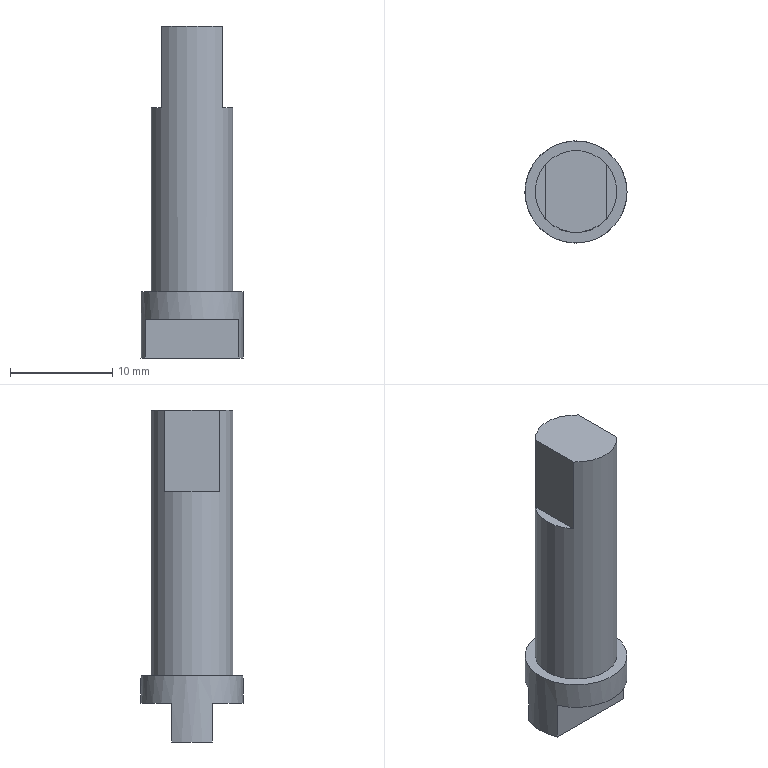Component | NX | VALVE_STEM | 1 solid | 13 faces | box 10 x 10 x 32.5 mm | volume 1609 mm3 | plane 11 | cylinder 2 | commonest cylinder face diameters 10 x1 8 x1
STEP:
#1=CARTESIAN_POINT('',(0.,0.,0.));
#2=DIRECTION('',(0.,0.,1.));
#3=DIRECTION('',(1.,0.,0.));
#4=AXIS2_PLACEMENT_3D('',#1,#2,#3);
#5=CARTESIAN_POINT('',(4.,14.,37.2));
#6=VERTEX_POINT('',#5);
#7=CARTESIAN_POINT('',(0.,14.,37.2));
#8=DIRECTION('',(0.,0.,1.));
#9=DIRECTION('',(1.,0.,0.));
#10=AXIS2_PLACEMENT_3D('',#7,#8,#9);
#11=CIRCLE('',#10,4.);
#12=CARTESIAN_POINT('',(0.,14.,37.2));
#13=DIRECTION('',(0.,0.,1.));
#14=DIRECTION('',(1.,0.,0.));
#15=AXIS2_PLACEMENT_3D('',#12,#13,#14);
#16=PLANE('',#15);
#17=CARTESIAN_POINT('',(0.,0.));
#18=DIRECTION('',(1.,0.));
#19=AXIS2_PLACEMENT_2D('',#17,#18);
#20=CIRCLE('',#19,4.);
#21=(GEOMETRIC_REPRESENTATION_CONTEXT(2)PARAMETRIC_REPRESENTATION_CONTEXT()REPRESENTATION_CONTEXT('',''));
#22=DEFINITIONAL_REPRESENTATION('',(#20),#21);
#23=PCURVE('',#16,#22);
#24=CARTESIAN_POINT('',(0.,14.,37.2));
#25=DIRECTION('',(0.,0.,1.));
#26=DIRECTION('',(1.,0.,0.));
#27=AXIS2_PLACEMENT_3D('',#24,#25,#26);
#28=CYLINDRICAL_SURFACE('',#27,4.);
#29=CARTESIAN_POINT('',(0.,0.));
#30=DIRECTION('',(1.,0.));
#31=VECTOR('',#30,1.);
#32=LINE('',#29,#31);
#33=(GEOMETRIC_REPRESENTATION_CONTEXT(2)PARAMETRIC_REPRESENTATION_CONTEXT()REPRESENTATION_CONTEXT('',''));
#34=DEFINITIONAL_REPRESENTATION('',(#32),#33);
#35=PCURVE('',#28,#34);
#36=SURFACE_CURVE('',#11,(#23,#35),.PCURVE_S1.);
#37=EDGE_CURVE('',#6,#6,#36,.T.);
#38=ORIENTED_EDGE('',*,*,#37,.F.);
#39=EDGE_LOOP('',(#38));
#40=FACE_BOUND('',#39,.T.);
#41=CARTESIAN_POINT('',(5.,14.,37.2));
#42=VERTEX_POINT('',#41);
#43=CARTESIAN_POINT('',(0.,14.,37.2));
#44=DIRECTION('',(0.,0.,-1.));
#45=DIRECTION('',(1.,0.,0.));
#46=AXIS2_PLACEMENT_3D('',#43,#44,#45);
#47=CIRCLE('',#46,5.);
#48=CARTESIAN_POINT('',(5.,0.));
#49=CARTESIAN_POINT('',(5.,-8.66));
#50=CARTESIAN_POINT('',(-2.5,-4.33));
#51=CARTESIAN_POINT('',(-10.,-0.));
#52=CARTESIAN_POINT('',(-2.5,4.33));
#53=CARTESIAN_POINT('',(5.,8.66));
#54=CARTESIAN_POINT('',(5.,0.));
#55=(BOUNDED_CURVE()B_SPLINE_CURVE(2,(#48,#49,#50,#51,#52,#53,#54),.UNSPECIFIED.,.T.,.F.)B_SPLINE_CURVE_WITH_KNOTS((1,2,2,2,2,1),(-2.094,0.,2.094,4.189,6.283,8.378),.UNSPECIFIED.)CURVE()GEOMETRIC_REPRESENTATION_ITEM()RATIONAL_B_SPLINE_CURVE((1.,0.5,1.,0.5,1.,0.5,1.))REPRESENTATION_ITEM(''));
#56=(GEOMETRIC_REPRESENTATION_CONTEXT(2)PARAMETRIC_REPRESENTATION_CONTEXT()REPRESENTATION_CONTEXT('',''));
#57=DEFINITIONAL_REPRESENTATION('',(#55),#56);
#58=PCURVE('',#16,#57);
#59=CARTESIAN_POINT('',(0.,14.,30.7));
#60=DIRECTION('',(0.,0.,1.));
#61=DIRECTION('',(1.,0.,0.));
#62=AXIS2_PLACEMENT_3D('',#59,#60,#61);
#63=CYLINDRICAL_SURFACE('',#62,5.);
#64=CARTESIAN_POINT('',(6.283,6.5));
#65=DIRECTION('',(-1.,0.));
#66=VECTOR('',#65,1.);
#67=LINE('',#64,#66);
#68=(GEOMETRIC_REPRESENTATION_CONTEXT(2)PARAMETRIC_REPRESENTATION_CONTEXT()REPRESENTATION_CONTEXT('',''));
#69=DEFINITIONAL_REPRESENTATION('',(#67),#68);
#70=PCURVE('',#63,#69);
#71=SURFACE_CURVE('',#47,(#58,#70),.PCURVE_S1.);
#72=EDGE_CURVE('',#42,#42,#71,.T.);
#73=ORIENTED_EDGE('',*,*,#72,.F.);
#74=EDGE_LOOP('',(#73));
#75=FACE_BOUND('',#74,.T.);
#76=ADVANCED_FACE('',(#40,#75),#16,.T.);
#77=CARTESIAN_POINT('',(-4.583,12.,30.7));
#78=VERTEX_POINT('',#77);
#79=CARTESIAN_POINT('',(4.583,12.,30.7));
#80=VERTEX_POINT('',#79);
#81=CARTESIAN_POINT('',(0.,12.,30.7));
#82=DIRECTION('',(1.,0.,0.));
#83=VECTOR('',#82,1.);
#84=LINE('',#81,#83);
#85=CARTESIAN_POINT('',(0.,14.,30.7));
#86=DIRECTION('',(0.,0.,-1.));
#87=DIRECTION('',(-1.,0.,0.));
#88=AXIS2_PLACEMENT_3D('',#85,#86,#87);
#89=PLANE('',#88);
#90=CARTESIAN_POINT('',(0.,-2.));
#91=DIRECTION('',(-1.,0.));
#92=VECTOR('',#91,1.);
#93=LINE('',#90,#92);
#94=(GEOMETRIC_REPRESENTATION_CONTEXT(2)PARAMETRIC_REPRESENTATION_CONTEXT()REPRESENTATION_CONTEXT('',''));
#95=DEFINITIONAL_REPRESENTATION('',(#93),#94);
#96=PCURVE('',#89,#95);
#97=CARTESIAN_POINT('',(-10.,12.,29.7));
#98=DIRECTION('',(0.,1.,-0.));
#99=DIRECTION('',(0.,0.,1.));
#100=AXIS2_PLACEMENT_3D('',#97,#98,#99);
#101=PLANE('',#100);
#102=CARTESIAN_POINT('',(1.,10.));
#103=DIRECTION('',(0.,1.));
#104=VECTOR('',#103,1.);
#105=LINE('',#102,#104);
#106=(GEOMETRIC_REPRESENTATION_CONTEXT(2)PARAMETRIC_REPRESENTATION_CONTEXT()REPRESENTATION_CONTEXT('',''));
#107=DEFINITIONAL_REPRESENTATION('',(#105),#106);
#108=PCURVE('',#101,#107);
#109=SURFACE_CURVE('',#84,(#96,#108),.PCURVE_S1.);
#110=EDGE_CURVE('',#78,#80,#109,.T.);
#111=ORIENTED_EDGE('',*,*,#110,.F.);
#112=CARTESIAN_POINT('',(-4.583,16.,30.7));
#113=VERTEX_POINT('',#112);
#114=CARTESIAN_POINT('',(0.,14.,30.7));
#115=DIRECTION('',(0.,0.,1.));
#116=DIRECTION('',(1.,0.,0.));
#117=AXIS2_PLACEMENT_3D('',#114,#115,#116);
#118=CIRCLE('',#117,5.);
#119=CARTESIAN_POINT('',(-5.,0.));
#120=CARTESIAN_POINT('',(-5.,8.66));
#121=CARTESIAN_POINT('',(2.5,4.33));
#122=CARTESIAN_POINT('',(10.,0.));
#123=CARTESIAN_POINT('',(2.5,-4.33));
#124=CARTESIAN_POINT('',(-5.,-8.66));
#125=CARTESIAN_POINT('',(-5.,0.));
#126=(BOUNDED_CURVE()B_SPLINE_CURVE(2,(#119,#120,#121,#122,#123,#124,#125),.UNSPECIFIED.,.T.,.F.)B_SPLINE_CURVE_WITH_KNOTS((1,2,2,2,2,1),(-2.094,0.,2.094,4.189,6.283,8.378),.UNSPECIFIED.)CURVE()GEOMETRIC_REPRESENTATION_ITEM()RATIONAL_B_SPLINE_CURVE((1.,0.5,1.,0.5,1.,0.5,1.))REPRESENTATION_ITEM(''));
#127=(GEOMETRIC_REPRESENTATION_CONTEXT(2)PARAMETRIC_REPRESENTATION_CONTEXT()REPRESENTATION_CONTEXT('',''));
#128=DEFINITIONAL_REPRESENTATION('',(#126),#127);
#129=PCURVE('',#89,#128);
#130=CARTESIAN_POINT('',(0.,0.));
#131=DIRECTION('',(1.,0.));
#132=VECTOR('',#131,1.);
#133=LINE('',#130,#132);
#134=(GEOMETRIC_REPRESENTATION_CONTEXT(2)PARAMETRIC_REPRESENTATION_CONTEXT()REPRESENTATION_CONTEXT('',''));
#135=DEFINITIONAL_REPRESENTATION('',(#133),#134);
#136=PCURVE('',#63,#135);
#137=SURFACE_CURVE('',#118,(#129,#136),.PCURVE_S1.);
#138=EDGE_CURVE('',#113,#78,#137,.T.);
#139=ORIENTED_EDGE('',*,*,#138,.F.);
#140=CARTESIAN_POINT('',(4.583,16.,30.7));
#141=VERTEX_POINT('',#140);
#142=CARTESIAN_POINT('',(0.,16.,30.7));
#143=DIRECTION('',(-1.,0.,0.));
#144=VECTOR('',#143,1.);
#145=LINE('',#142,#144);
#146=CARTESIAN_POINT('',(0.,2.));
#147=DIRECTION('',(1.,0.));
#148=VECTOR('',#147,1.);
#149=LINE('',#146,#148);
#150=(GEOMETRIC_REPRESENTATION_CONTEXT(2)PARAMETRIC_REPRESENTATION_CONTEXT()REPRESENTATION_CONTEXT('',''));
#151=DEFINITIONAL_REPRESENTATION('',(#149),#150);
#152=PCURVE('',#89,#151);
#153=CARTESIAN_POINT('',(-10.,16.,34.5));
#154=DIRECTION('',(0.,-1.,-0.));
#155=DIRECTION('',(0.,0.,-1.));
#156=AXIS2_PLACEMENT_3D('',#153,#154,#155);
#157=PLANE('',#156);
#158=CARTESIAN_POINT('',(3.8,10.));
#159=DIRECTION('',(0.,-1.));
#160=VECTOR('',#159,1.);
#161=LINE('',#158,#160);
#162=(GEOMETRIC_REPRESENTATION_CONTEXT(2)PARAMETRIC_REPRESENTATION_CONTEXT()REPRESENTATION_CONTEXT('',''));
#163=DEFINITIONAL_REPRESENTATION('',(#161),#162);
#164=PCURVE('',#157,#163);
#165=SURFACE_CURVE('',#145,(#152,#164),.PCURVE_S1.);
#166=EDGE_CURVE('',#141,#113,#165,.T.);
#167=ORIENTED_EDGE('',*,*,#166,.F.);
#168=CARTESIAN_POINT('',(5.,14.,30.7));
#169=VERTEX_POINT('',#168);
#170=CARTESIAN_POINT('',(0.,14.,30.7));
#171=DIRECTION('',(0.,0.,1.));
#172=DIRECTION('',(1.,0.,0.));
#173=AXIS2_PLACEMENT_3D('',#170,#171,#172);
#174=CIRCLE('',#173,5.);
#175=CARTESIAN_POINT('',(-5.,0.));
#176=CARTESIAN_POINT('',(-5.,8.66));
#177=CARTESIAN_POINT('',(2.5,4.33));
#178=CARTESIAN_POINT('',(10.,0.));
#179=CARTESIAN_POINT('',(2.5,-4.33));
#180=CARTESIAN_POINT('',(-5.,-8.66));
#181=CARTESIAN_POINT('',(-5.,0.));
#182=(BOUNDED_CURVE()B_SPLINE_CURVE(2,(#175,#176,#177,#178,#179,#180,#181),.UNSPECIFIED.,.T.,.F.)B_SPLINE_CURVE_WITH_KNOTS((1,2,2,2,2,1),(-2.094,0.,2.094,4.189,6.283,8.378),.UNSPECIFIED.)CURVE()GEOMETRIC_REPRESENTATION_ITEM()RATIONAL_B_SPLINE_CURVE((1.,0.5,1.,0.5,1.,0.5,1.))REPRESENTATION_ITEM(''));
#183=(GEOMETRIC_REPRESENTATION_CONTEXT(2)PARAMETRIC_REPRESENTATION_CONTEXT()REPRESENTATION_CONTEXT('',''));
#184=DEFINITIONAL_REPRESENTATION('',(#182),#183);
#185=PCURVE('',#89,#184);
#186=CARTESIAN_POINT('',(-6.283,0.));
#187=DIRECTION('',(1.,0.));
#188=VECTOR('',#187,1.);
#189=LINE('',#186,#188);
#190=(GEOMETRIC_REPRESENTATION_CONTEXT(2)PARAMETRIC_REPRESENTATION_CONTEXT()REPRESENTATION_CONTEXT('',''));
#191=DEFINITIONAL_REPRESENTATION('',(#189),#190);
#192=PCURVE('',#63,#191);
#193=SURFACE_CURVE('',#174,(#185,#192),.PCURVE_S1.);
#194=EDGE_CURVE('',#169,#141,#193,.T.);
#195=ORIENTED_EDGE('',*,*,#194,.F.);
#196=CARTESIAN_POINT('',(0.,14.,30.7));
#197=DIRECTION('',(0.,0.,1.));
#198=DIRECTION('',(1.,0.,0.));
#199=AXIS2_PLACEMENT_3D('',#196,#197,#198);
#200=CIRCLE('',#199,5.);
#201=CARTESIAN_POINT('',(-5.,0.));
#202=CARTESIAN_POINT('',(-5.,8.66));
#203=CARTESIAN_POINT('',(2.5,4.33));
#204=CARTESIAN_POINT('',(10.,0.));
#205=CARTESIAN_POINT('',(2.5,-4.33));
#206=CARTESIAN_POINT('',(-5.,-8.66));
#207=CARTESIAN_POINT('',(-5.,0.));
#208=(BOUNDED_CURVE()B_SPLINE_CURVE(2,(#201,#202,#203,#204,#205,#206,#207),.UNSPECIFIED.,.T.,.F.)B_SPLINE_CURVE_WITH_KNOTS((1,2,2,2,2,1),(-2.094,0.,2.094,4.189,6.283,8.378),.UNSPECIFIED.)CURVE()GEOMETRIC_REPRESENTATION_ITEM()RATIONAL_B_SPLINE_CURVE((1.,0.5,1.,0.5,1.,0.5,1.))REPRESENTATION_ITEM(''));
#209=(GEOMETRIC_REPRESENTATION_CONTEXT(2)PARAMETRIC_REPRESENTATION_CONTEXT()REPRESENTATION_CONTEXT('',''));
#210=DEFINITIONAL_REPRESENTATION('',(#208),#209);
#211=PCURVE('',#89,#210);
#212=CARTESIAN_POINT('',(0.,0.));
#213=DIRECTION('',(1.,0.));
#214=VECTOR('',#213,1.);
#215=LINE('',#212,#214);
#216=(GEOMETRIC_REPRESENTATION_CONTEXT(2)PARAMETRIC_REPRESENTATION_CONTEXT()REPRESENTATION_CONTEXT('',''));
#217=DEFINITIONAL_REPRESENTATION('',(#215),#216);
#218=PCURVE('',#63,#217);
#219=SURFACE_CURVE('',#200,(#211,#218),.PCURVE_S1.);
#220=EDGE_CURVE('',#80,#169,#219,.T.);
#221=ORIENTED_EDGE('',*,*,#220,.F.);
#222=EDGE_LOOP('',(#111,#139,#167,#195,#221));
#223=FACE_BOUND('',#222,.T.);
#224=ADVANCED_FACE('',(#223),#89,.T.);
#225=CARTESIAN_POINT('',(-4.583,12.,34.5));
#226=VERTEX_POINT('',#225);
#227=CARTESIAN_POINT('',(-4.583,12.,30.7));
#228=DIRECTION('',(0.,0.,-1.));
#229=VECTOR('',#228,1.);
#230=LINE('',#227,#229);
#231=CARTESIAN_POINT('',(3.553,0.));
#232=DIRECTION('',(0.,-1.));
#233=VECTOR('',#232,1.);
#234=LINE('',#231,#233);
#235=(GEOMETRIC_REPRESENTATION_CONTEXT(2)PARAMETRIC_REPRESENTATION_CONTEXT()REPRESENTATION_CONTEXT('',''));
#236=DEFINITIONAL_REPRESENTATION('',(#234),#235);
#237=PCURVE('',#63,#236);
#238=CARTESIAN_POINT('',(1.,5.417));
#239=DIRECTION('',(-1.,0.));
#240=VECTOR('',#239,1.);
#241=LINE('',#238,#240);
#242=(GEOMETRIC_REPRESENTATION_CONTEXT(2)PARAMETRIC_REPRESENTATION_CONTEXT()REPRESENTATION_CONTEXT('',''));
#243=DEFINITIONAL_REPRESENTATION('',(#241),#242);
#244=PCURVE('',#101,#243);
#245=SURFACE_CURVE('',#230,(#237,#244),.PCURVE_S1.);
#246=EDGE_CURVE('',#226,#78,#245,.T.);
#247=ORIENTED_EDGE('',*,*,#246,.F.);
#248=CARTESIAN_POINT('',(4.583,12.,34.5));
#249=VERTEX_POINT('',#248);
#250=CARTESIAN_POINT('',(0.,14.,34.5));
#251=DIRECTION('',(0.,0.,-1.));
#252=DIRECTION('',(1.,0.,0.));
#253=AXIS2_PLACEMENT_3D('',#250,#251,#252);
#254=CIRCLE('',#253,5.);
#255=CARTESIAN_POINT('',(6.283,3.8));
#256=DIRECTION('',(-1.,0.));
#257=VECTOR('',#256,1.);
#258=LINE('',#255,#257);
#259=(GEOMETRIC_REPRESENTATION_CONTEXT(2)PARAMETRIC_REPRESENTATION_CONTEXT()REPRESENTATION_CONTEXT('',''));
#260=DEFINITIONAL_REPRESENTATION('',(#258),#259);
#261=PCURVE('',#63,#260);
#262=CARTESIAN_POINT('',(-10.,12.,34.5));
#263=DIRECTION('',(0.,0.,1.));
#264=DIRECTION('',(1.,0.,0.));
#265=AXIS2_PLACEMENT_3D('',#262,#263,#264);
#266=PLANE('',#265);
#267=CARTESIAN_POINT('',(15.,2.));
#268=CARTESIAN_POINT('',(15.,-6.66));
#269=CARTESIAN_POINT('',(7.5,-2.33));
#270=CARTESIAN_POINT('',(0.,2.));
#271=CARTESIAN_POINT('',(7.5,6.33));
#272=CARTESIAN_POINT('',(15.,10.66));
#273=CARTESIAN_POINT('',(15.,2.));
#274=(BOUNDED_CURVE()B_SPLINE_CURVE(2,(#267,#268,#269,#270,#271,#272,#273),.UNSPECIFIED.,.T.,.F.)B_SPLINE_CURVE_WITH_KNOTS((1,2,2,2,2,1),(-2.094,0.,2.094,4.189,6.283,8.378),.UNSPECIFIED.)CURVE()GEOMETRIC_REPRESENTATION_ITEM()RATIONAL_B_SPLINE_CURVE((1.,0.5,1.,0.5,1.,0.5,1.))REPRESENTATION_ITEM(''));
#275=(GEOMETRIC_REPRESENTATION_CONTEXT(2)PARAMETRIC_REPRESENTATION_CONTEXT()REPRESENTATION_CONTEXT('',''));
#276=DEFINITIONAL_REPRESENTATION('',(#274),#275);
#277=PCURVE('',#266,#276);
#278=SURFACE_CURVE('',#254,(#261,#277),.PCURVE_S1.);
#279=EDGE_CURVE('',#249,#226,#278,.T.);
#280=ORIENTED_EDGE('',*,*,#279,.F.);
#281=CARTESIAN_POINT('',(4.583,12.,30.7));
#282=DIRECTION('',(0.,0.,1.));
#283=VECTOR('',#282,1.);
#284=LINE('',#281,#283);
#285=CARTESIAN_POINT('',(5.872,0.));
#286=DIRECTION('',(0.,1.));
#287=VECTOR('',#286,1.);
#288=LINE('',#285,#287);
#289=(GEOMETRIC_REPRESENTATION_CONTEXT(2)PARAMETRIC_REPRESENTATION_CONTEXT()REPRESENTATION_CONTEXT('',''));
#290=DEFINITIONAL_REPRESENTATION('',(#288),#289);
#291=PCURVE('',#63,#290);
#292=CARTESIAN_POINT('',(1.,14.583));
#293=DIRECTION('',(1.,0.));
#294=VECTOR('',#293,1.);
#295=LINE('',#292,#294);
#296=(GEOMETRIC_REPRESENTATION_CONTEXT(2)PARAMETRIC_REPRESENTATION_CONTEXT()REPRESENTATION_CONTEXT('',''));
#297=DEFINITIONAL_REPRESENTATION('',(#295),#296);
#298=PCURVE('',#101,#297);
#299=SURFACE_CURVE('',#284,(#291,#298),.PCURVE_S1.);
#300=EDGE_CURVE('',#80,#249,#299,.T.);
#301=ORIENTED_EDGE('',*,*,#300,.F.);
#302=ORIENTED_EDGE('',*,*,#220,.T.);
#303=CARTESIAN_POINT('',(5.,14.,30.7));
#304=CARTESIAN_POINT('',(5.,14.,37.2));
#305=B_SPLINE_CURVE_WITH_KNOTS('',1,(#303,#304),.UNSPECIFIED.,.F.,.F.,(2,2),(0.,6.5),.PIECEWISE_BEZIER_KNOTS.);
#306=CARTESIAN_POINT('',(6.283,0.));
#307=DIRECTION('',(0.,1.));
#308=VECTOR('',#307,1.);
#309=LINE('',#306,#308);
#310=(GEOMETRIC_REPRESENTATION_CONTEXT(2)PARAMETRIC_REPRESENTATION_CONTEXT()REPRESENTATION_CONTEXT('',''));
#311=DEFINITIONAL_REPRESENTATION('',(#309),#310);
#312=PCURVE('',#63,#311);
#313=CARTESIAN_POINT('',(0.,0.));
#314=DIRECTION('',(0.,1.));
#315=VECTOR('',#314,1.);
#316=LINE('',#313,#315);
#317=(GEOMETRIC_REPRESENTATION_CONTEXT(2)PARAMETRIC_REPRESENTATION_CONTEXT()REPRESENTATION_CONTEXT('',''));
#318=DEFINITIONAL_REPRESENTATION('',(#316),#317);
#319=PCURVE('',#63,#318);
#320=SEAM_CURVE('',#305,(#312,#319),.PCURVE_S1.);
#321=EDGE_CURVE('',#169,#42,#320,.T.);
#322=ORIENTED_EDGE('',*,*,#321,.T.);
#323=ORIENTED_EDGE('',*,*,#72,.T.);
#324=ORIENTED_EDGE('',*,*,#321,.F.);
#325=ORIENTED_EDGE('',*,*,#194,.T.);
#326=CARTESIAN_POINT('',(4.583,16.,34.5));
#327=VERTEX_POINT('',#326);
#328=CARTESIAN_POINT('',(4.583,16.,30.7));
#329=DIRECTION('',(0.,0.,-1.));
#330=VECTOR('',#329,1.);
#331=LINE('',#328,#330);
#332=CARTESIAN_POINT('',(0.4115,0.));
#333=DIRECTION('',(0.,-1.));
#334=VECTOR('',#333,1.);
#335=LINE('',#332,#334);
#336=(GEOMETRIC_REPRESENTATION_CONTEXT(2)PARAMETRIC_REPRESENTATION_CONTEXT()REPRESENTATION_CONTEXT('',''));
#337=DEFINITIONAL_REPRESENTATION('',(#335),#336);
#338=PCURVE('',#63,#337);
#339=CARTESIAN_POINT('',(3.8,14.583));
#340=DIRECTION('',(1.,0.));
#341=VECTOR('',#340,1.);
#342=LINE('',#339,#341);
#343=(GEOMETRIC_REPRESENTATION_CONTEXT(2)PARAMETRIC_REPRESENTATION_CONTEXT()REPRESENTATION_CONTEXT('',''));
#344=DEFINITIONAL_REPRESENTATION('',(#342),#343);
#345=PCURVE('',#157,#344);
#346=SURFACE_CURVE('',#331,(#338,#345),.PCURVE_S1.);
#347=EDGE_CURVE('',#327,#141,#346,.T.);
#348=ORIENTED_EDGE('',*,*,#347,.F.);
#349=CARTESIAN_POINT('',(-4.583,16.,34.5));
#350=VERTEX_POINT('',#349);
#351=CARTESIAN_POINT('',(0.,14.,34.5));
#352=DIRECTION('',(0.,0.,-1.));
#353=DIRECTION('',(1.,0.,0.));
#354=AXIS2_PLACEMENT_3D('',#351,#352,#353);
#355=CIRCLE('',#354,5.);
#356=CARTESIAN_POINT('',(6.283,3.8));
#357=DIRECTION('',(-1.,0.));
#358=VECTOR('',#357,1.);
#359=LINE('',#356,#358);
#360=(GEOMETRIC_REPRESENTATION_CONTEXT(2)PARAMETRIC_REPRESENTATION_CONTEXT()REPRESENTATION_CONTEXT('',''));
#361=DEFINITIONAL_REPRESENTATION('',(#359),#360);
#362=PCURVE('',#63,#361);
#363=CARTESIAN_POINT('',(-10.,22.,34.5));
#364=DIRECTION('',(0.,0.,1.));
#365=DIRECTION('',(1.,0.,0.));
#366=AXIS2_PLACEMENT_3D('',#363,#364,#365);
#367=PLANE('',#366);
#368=CARTESIAN_POINT('',(15.,-8.));
#369=CARTESIAN_POINT('',(15.,-16.66));
#370=CARTESIAN_POINT('',(7.5,-12.33));
#371=CARTESIAN_POINT('',(0.,-8.));
#372=CARTESIAN_POINT('',(7.5,-3.67));
#373=CARTESIAN_POINT('',(15.,0.6603));
#374=CARTESIAN_POINT('',(15.,-8.));
#375=(BOUNDED_CURVE()B_SPLINE_CURVE(2,(#368,#369,#370,#371,#372,#373,#374),.UNSPECIFIED.,.T.,.F.)B_SPLINE_CURVE_WITH_KNOTS((1,2,2,2,2,1),(-2.094,0.,2.094,4.189,6.283,8.378),.UNSPECIFIED.)CURVE()GEOMETRIC_REPRESENTATION_ITEM()RATIONAL_B_SPLINE_CURVE((1.,0.5,1.,0.5,1.,0.5,1.))REPRESENTATION_ITEM(''));
#376=(GEOMETRIC_REPRESENTATION_CONTEXT(2)PARAMETRIC_REPRESENTATION_CONTEXT()REPRESENTATION_CONTEXT('',''));
#377=DEFINITIONAL_REPRESENTATION('',(#375),#376);
#378=PCURVE('',#367,#377);
#379=SURFACE_CURVE('',#355,(#362,#378),.PCURVE_S1.);
#380=EDGE_CURVE('',#350,#327,#379,.T.);
#381=ORIENTED_EDGE('',*,*,#380,.F.);
#382=CARTESIAN_POINT('',(-4.583,16.,30.7));
#383=DIRECTION('',(0.,0.,1.));
#384=VECTOR('',#383,1.);
#385=LINE('',#382,#384);
#386=CARTESIAN_POINT('',(2.73,0.));
#387=DIRECTION('',(0.,1.));
#388=VECTOR('',#387,1.);
#389=LINE('',#386,#388);
#390=(GEOMETRIC_REPRESENTATION_CONTEXT(2)PARAMETRIC_REPRESENTATION_CONTEXT()REPRESENTATION_CONTEXT('',''));
#391=DEFINITIONAL_REPRESENTATION('',(#389),#390);
#392=PCURVE('',#63,#391);
#393=CARTESIAN_POINT('',(3.8,5.417));
#394=DIRECTION('',(-1.,0.));
#395=VECTOR('',#394,1.);
#396=LINE('',#393,#395);
#397=(GEOMETRIC_REPRESENTATION_CONTEXT(2)PARAMETRIC_REPRESENTATION_CONTEXT()REPRESENTATION_CONTEXT('',''));
#398=DEFINITIONAL_REPRESENTATION('',(#396),#397);
#399=PCURVE('',#157,#398);
#400=SURFACE_CURVE('',#385,(#392,#399),.PCURVE_S1.);
#401=EDGE_CURVE('',#113,#350,#400,.T.);
#402=ORIENTED_EDGE('',*,*,#401,.F.);
#403=ORIENTED_EDGE('',*,*,#138,.T.);
#404=EDGE_LOOP('',(#247,#280,#301,#302,#322,#323,#324,#325,#348,#381,#402,#403));
#405=FACE_BOUND('',#404,.T.);
#406=ADVANCED_FACE('',(#405),#63,.T.);
#407=CARTESIAN_POINT('',(-3.,11.354,63.2));
#408=VERTEX_POINT('',#407);
#409=CARTESIAN_POINT('',(-3.,16.646,63.2));
#410=VERTEX_POINT('',#409);
#411=CARTESIAN_POINT('',(-3.,9.7,63.2));
#412=DIRECTION('',(0.,1.,0.));
#413=VECTOR('',#412,1.);
#414=LINE('',#411,#413);
#415=CARTESIAN_POINT('',(0.,14.,63.2));
#416=DIRECTION('',(0.,0.,1.));
#417=DIRECTION('',(1.,0.,0.));
#418=AXIS2_PLACEMENT_3D('',#415,#416,#417);
#419=PLANE('',#418);
#420=CARTESIAN_POINT('',(-3.,-4.3));
#421=DIRECTION('',(0.,1.));
#422=VECTOR('',#421,1.);
#423=LINE('',#420,#422);
#424=(GEOMETRIC_REPRESENTATION_CONTEXT(2)PARAMETRIC_REPRESENTATION_CONTEXT()REPRESENTATION_CONTEXT('',''));
#425=DEFINITIONAL_REPRESENTATION('',(#423),#424);
#426=PCURVE('',#419,#425);
#427=CARTESIAN_POINT('',(-3.,9.7,55.2));
#428=DIRECTION('',(1.,-0.,0.));
#429=DIRECTION('',(0.,1.,0.));
#430=AXIS2_PLACEMENT_3D('',#427,#428,#429);
#431=PLANE('',#430);
#432=CARTESIAN_POINT('',(0.,8.));
#433=DIRECTION('',(1.,0.));
#434=VECTOR('',#433,1.);
#435=LINE('',#432,#434);
#436=(GEOMETRIC_REPRESENTATION_CONTEXT(2)PARAMETRIC_REPRESENTATION_CONTEXT()REPRESENTATION_CONTEXT('',''));
#437=DEFINITIONAL_REPRESENTATION('',(#435),#436);
#438=PCURVE('',#431,#437);
#439=SURFACE_CURVE('',#414,(#426,#438),.PCURVE_S1.);
#440=EDGE_CURVE('',#408,#410,#439,.T.);
#441=ORIENTED_EDGE('',*,*,#440,.F.);
#442=CARTESIAN_POINT('',(3.,11.354,63.2));
#443=VERTEX_POINT('',#442);
#444=CARTESIAN_POINT('',(0.,14.,63.2));
#445=DIRECTION('',(0.,0.,-1.));
#446=DIRECTION('',(1.,0.,0.));
#447=AXIS2_PLACEMENT_3D('',#444,#445,#446);
#448=CIRCLE('',#447,4.);
#449=CARTESIAN_POINT('',(4.,0.));
#450=CARTESIAN_POINT('',(4.,-6.928));
#451=CARTESIAN_POINT('',(-2.,-3.464));
#452=CARTESIAN_POINT('',(-8.,-0.));
#453=CARTESIAN_POINT('',(-2.,3.464));
#454=CARTESIAN_POINT('',(4.,6.928));
#455=CARTESIAN_POINT('',(4.,0.));
#456=(BOUNDED_CURVE()B_SPLINE_CURVE(2,(#449,#450,#451,#452,#453,#454,#455),.UNSPECIFIED.,.T.,.F.)B_SPLINE_CURVE_WITH_KNOTS((1,2,2,2,2,1),(-2.094,0.,2.094,4.189,6.283,8.378),.UNSPECIFIED.)CURVE()GEOMETRIC_REPRESENTATION_ITEM()RATIONAL_B_SPLINE_CURVE((1.,0.5,1.,0.5,1.,0.5,1.))REPRESENTATION_ITEM(''));
#457=(GEOMETRIC_REPRESENTATION_CONTEXT(2)PARAMETRIC_REPRESENTATION_CONTEXT()REPRESENTATION_CONTEXT('',''));
#458=DEFINITIONAL_REPRESENTATION('',(#456),#457);
#459=PCURVE('',#419,#458);
#460=CARTESIAN_POINT('',(6.283,26.));
#461=DIRECTION('',(-1.,0.));
#462=VECTOR('',#461,1.);
#463=LINE('',#460,#462);
#464=(GEOMETRIC_REPRESENTATION_CONTEXT(2)PARAMETRIC_REPRESENTATION_CONTEXT()REPRESENTATION_CONTEXT('',''));
#465=DEFINITIONAL_REPRESENTATION('',(#463),#464);
#466=PCURVE('',#28,#465);
#467=SURFACE_CURVE('',#448,(#459,#466),.PCURVE_S1.);
#468=EDGE_CURVE('',#443,#408,#467,.T.);
#469=ORIENTED_EDGE('',*,*,#468,.F.);
#470=CARTESIAN_POINT('',(3.,16.646,63.2));
#471=VERTEX_POINT('',#470);
#472=CARTESIAN_POINT('',(3.,19.4,63.2));
#473=DIRECTION('',(0.,-1.,0.));
#474=VECTOR('',#473,1.);
#475=LINE('',#472,#474);
#476=CARTESIAN_POINT('',(3.,5.4));
#477=DIRECTION('',(0.,-1.));
#478=VECTOR('',#477,1.);
#479=LINE('',#476,#478);
#480=(GEOMETRIC_REPRESENTATION_CONTEXT(2)PARAMETRIC_REPRESENTATION_CONTEXT()REPRESENTATION_CONTEXT('',''));
#481=DEFINITIONAL_REPRESENTATION('',(#479),#480);
#482=PCURVE('',#419,#481);
#483=CARTESIAN_POINT('',(3.,19.4,55.2));
#484=DIRECTION('',(-1.,-0.,0.));
#485=DIRECTION('',(0.,-1.,0.));
#486=AXIS2_PLACEMENT_3D('',#483,#484,#485);
#487=PLANE('',#486);
#488=CARTESIAN_POINT('',(0.,8.));
#489=DIRECTION('',(1.,0.));
#490=VECTOR('',#489,1.);
#491=LINE('',#488,#490);
#492=(GEOMETRIC_REPRESENTATION_CONTEXT(2)PARAMETRIC_REPRESENTATION_CONTEXT()REPRESENTATION_CONTEXT('',''));
#493=DEFINITIONAL_REPRESENTATION('',(#491),#492);
#494=PCURVE('',#487,#493);
#495=SURFACE_CURVE('',#475,(#482,#494),.PCURVE_S1.);
#496=EDGE_CURVE('',#471,#443,#495,.T.);
#497=ORIENTED_EDGE('',*,*,#496,.F.);
#498=CARTESIAN_POINT('',(0.,14.,63.2));
#499=DIRECTION('',(0.,0.,-1.));
#500=DIRECTION('',(1.,0.,0.));
#501=AXIS2_PLACEMENT_3D('',#498,#499,#500);
#502=CIRCLE('',#501,4.);
#503=CARTESIAN_POINT('',(4.,0.));
#504=CARTESIAN_POINT('',(4.,-6.928));
#505=CARTESIAN_POINT('',(-2.,-3.464));
#506=CARTESIAN_POINT('',(-8.,-0.));
#507=CARTESIAN_POINT('',(-2.,3.464));
#508=CARTESIAN_POINT('',(4.,6.928));
#509=CARTESIAN_POINT('',(4.,0.));
#510=(BOUNDED_CURVE()B_SPLINE_CURVE(2,(#503,#504,#505,#506,#507,#508,#509),.UNSPECIFIED.,.T.,.F.)B_SPLINE_CURVE_WITH_KNOTS((1,2,2,2,2,1),(-2.094,0.,2.094,4.189,6.283,8.378),.UNSPECIFIED.)CURVE()GEOMETRIC_REPRESENTATION_ITEM()RATIONAL_B_SPLINE_CURVE((1.,0.5,1.,0.5,1.,0.5,1.))REPRESENTATION_ITEM(''));
#511=(GEOMETRIC_REPRESENTATION_CONTEXT(2)PARAMETRIC_REPRESENTATION_CONTEXT()REPRESENTATION_CONTEXT('',''));
#512=DEFINITIONAL_REPRESENTATION('',(#510),#511);
#513=PCURVE('',#419,#512);
#514=CARTESIAN_POINT('',(6.283,26.));
#515=DIRECTION('',(-1.,0.));
#516=VECTOR('',#515,1.);
#517=LINE('',#514,#516);
#518=(GEOMETRIC_REPRESENTATION_CONTEXT(2)PARAMETRIC_REPRESENTATION_CONTEXT()REPRESENTATION_CONTEXT('',''));
#519=DEFINITIONAL_REPRESENTATION('',(#517),#518);
#520=PCURVE('',#28,#519);
#521=SURFACE_CURVE('',#502,(#513,#520),.PCURVE_S1.);
#522=EDGE_CURVE('',#410,#471,#521,.T.);
#523=ORIENTED_EDGE('',*,*,#522,.F.);
#524=EDGE_LOOP('',(#441,#469,#497,#523));
#525=FACE_BOUND('',#524,.T.);
#526=ADVANCED_FACE('',(#525),#419,.T.);
#527=CARTESIAN_POINT('',(-3.,16.646,55.2));
#528=VERTEX_POINT('',#527);
#529=CARTESIAN_POINT('',(-3.,16.646,37.2));
#530=DIRECTION('',(0.,0.,-1.));
#531=VECTOR('',#530,1.);
#532=LINE('',#529,#531);
#533=CARTESIAN_POINT('',(2.419,0.));
#534=DIRECTION('',(0.,-1.));
#535=VECTOR('',#534,1.);
#536=LINE('',#533,#535);
#537=(GEOMETRIC_REPRESENTATION_CONTEXT(2)PARAMETRIC_REPRESENTATION_CONTEXT()REPRESENTATION_CONTEXT('',''));
#538=DEFINITIONAL_REPRESENTATION('',(#536),#537);
#539=PCURVE('',#28,#538);
#540=CARTESIAN_POINT('',(6.946,-18.));
#541=DIRECTION('',(0.,-1.));
#542=VECTOR('',#541,1.);
#543=LINE('',#540,#542);
#544=(GEOMETRIC_REPRESENTATION_CONTEXT(2)PARAMETRIC_REPRESENTATION_CONTEXT()REPRESENTATION_CONTEXT('',''));
#545=DEFINITIONAL_REPRESENTATION('',(#543),#544);
#546=PCURVE('',#431,#545);
#547=SURFACE_CURVE('',#532,(#539,#546),.PCURVE_S1.);
#548=EDGE_CURVE('',#410,#528,#547,.T.);
#549=ORIENTED_EDGE('',*,*,#548,.F.);
#550=ORIENTED_EDGE('',*,*,#522,.T.);
#551=CARTESIAN_POINT('',(3.,16.646,55.2));
#552=VERTEX_POINT('',#551);
#553=CARTESIAN_POINT('',(3.,16.646,37.2));
#554=DIRECTION('',(0.,0.,1.));
#555=VECTOR('',#554,1.);
#556=LINE('',#553,#555);
#557=CARTESIAN_POINT('',(0.7227,0.));
#558=DIRECTION('',(0.,1.));
#559=VECTOR('',#558,1.);
#560=LINE('',#557,#559);
#561=(GEOMETRIC_REPRESENTATION_CONTEXT(2)PARAMETRIC_REPRESENTATION_CONTEXT()REPRESENTATION_CONTEXT('',''));
#562=DEFINITIONAL_REPRESENTATION('',(#560),#561);
#563=PCURVE('',#28,#562);
#564=CARTESIAN_POINT('',(2.754,-18.));
#565=DIRECTION('',(0.,1.));
#566=VECTOR('',#565,1.);
#567=LINE('',#564,#566);
#568=(GEOMETRIC_REPRESENTATION_CONTEXT(2)PARAMETRIC_REPRESENTATION_CONTEXT()REPRESENTATION_CONTEXT('',''));
#569=DEFINITIONAL_REPRESENTATION('',(#567),#568);
#570=PCURVE('',#487,#569);
#571=SURFACE_CURVE('',#556,(#563,#570),.PCURVE_S1.);
#572=EDGE_CURVE('',#552,#471,#571,.T.);
#573=ORIENTED_EDGE('',*,*,#572,.F.);
#574=CARTESIAN_POINT('',(4.,14.,55.2));
#575=VERTEX_POINT('',#574);
#576=CARTESIAN_POINT('',(0.,14.,55.2));
#577=DIRECTION('',(0.,0.,-1.));
#578=DIRECTION('',(1.,0.,0.));
#579=AXIS2_PLACEMENT_3D('',#576,#577,#578);
#580=CIRCLE('',#579,4.);
#581=CARTESIAN_POINT('',(6.283,18.));
#582=DIRECTION('',(-1.,0.));
#583=VECTOR('',#582,1.);
#584=LINE('',#581,#583);
#585=(GEOMETRIC_REPRESENTATION_CONTEXT(2)PARAMETRIC_REPRESENTATION_CONTEXT()REPRESENTATION_CONTEXT('',''));
#586=DEFINITIONAL_REPRESENTATION('',(#584),#585);
#587=PCURVE('',#28,#586);
#588=CARTESIAN_POINT('',(0.,14.,55.2));
#589=DIRECTION('',(0.,0.,1.));
#590=DIRECTION('',(1.,0.,0.));
#591=AXIS2_PLACEMENT_3D('',#588,#589,#590);
#592=PLANE('',#591);
#593=CARTESIAN_POINT('',(4.,0.));
#594=CARTESIAN_POINT('',(4.,-6.928));
#595=CARTESIAN_POINT('',(-2.,-3.464));
#596=CARTESIAN_POINT('',(-8.,-0.));
#597=CARTESIAN_POINT('',(-2.,3.464));
#598=CARTESIAN_POINT('',(4.,6.928));
#599=CARTESIAN_POINT('',(4.,0.));
#600=(BOUNDED_CURVE()B_SPLINE_CURVE(2,(#593,#594,#595,#596,#597,#598,#599),.UNSPECIFIED.,.T.,.F.)B_SPLINE_CURVE_WITH_KNOTS((1,2,2,2,2,1),(-2.094,0.,2.094,4.189,6.283,8.378),.UNSPECIFIED.)CURVE()GEOMETRIC_REPRESENTATION_ITEM()RATIONAL_B_SPLINE_CURVE((1.,0.5,1.,0.5,1.,0.5,1.))REPRESENTATION_ITEM(''));
#601=(GEOMETRIC_REPRESENTATION_CONTEXT(2)PARAMETRIC_REPRESENTATION_CONTEXT()REPRESENTATION_CONTEXT('',''));
#602=DEFINITIONAL_REPRESENTATION('',(#600),#601);
#603=PCURVE('',#592,#602);
#604=SURFACE_CURVE('',#580,(#587,#603),.PCURVE_S1.);
#605=EDGE_CURVE('',#552,#575,#604,.T.);
#606=ORIENTED_EDGE('',*,*,#605,.T.);
#607=CARTESIAN_POINT('',(4.,14.,37.2));
#608=CARTESIAN_POINT('',(4.,14.,55.2));
#609=B_SPLINE_CURVE_WITH_KNOTS('',1,(#607,#608),.UNSPECIFIED.,.F.,.F.,(2,2),(0.,18.),.PIECEWISE_BEZIER_KNOTS.);
#610=CARTESIAN_POINT('',(0.,0.));
#611=DIRECTION('',(0.,1.));
#612=VECTOR('',#611,1.);
#613=LINE('',#610,#612);
#614=(GEOMETRIC_REPRESENTATION_CONTEXT(2)PARAMETRIC_REPRESENTATION_CONTEXT()REPRESENTATION_CONTEXT('',''));
#615=DEFINITIONAL_REPRESENTATION('',(#613),#614);
#616=PCURVE('',#28,#615);
#617=CARTESIAN_POINT('',(6.283,0.));
#618=DIRECTION('',(0.,1.));
#619=VECTOR('',#618,1.);
#620=LINE('',#617,#619);
#621=(GEOMETRIC_REPRESENTATION_CONTEXT(2)PARAMETRIC_REPRESENTATION_CONTEXT()REPRESENTATION_CONTEXT('',''));
#622=DEFINITIONAL_REPRESENTATION('',(#620),#621);
#623=PCURVE('',#28,#622);
#624=SEAM_CURVE('',#609,(#616,#623),.PCURVE_S1.);
#625=EDGE_CURVE('',#6,#575,#624,.T.);
#626=ORIENTED_EDGE('',*,*,#625,.F.);
#627=ORIENTED_EDGE('',*,*,#37,.T.);
#628=ORIENTED_EDGE('',*,*,#625,.T.);
#629=CARTESIAN_POINT('',(3.,11.354,55.2));
#630=VERTEX_POINT('',#629);
#631=CARTESIAN_POINT('',(0.,14.,55.2));
#632=DIRECTION('',(0.,0.,-1.));
#633=DIRECTION('',(1.,0.,0.));
#634=AXIS2_PLACEMENT_3D('',#631,#632,#633);
#635=CIRCLE('',#634,4.);
#636=CARTESIAN_POINT('',(12.566,18.));
#637=DIRECTION('',(-1.,0.));
#638=VECTOR('',#637,1.);
#639=LINE('',#636,#638);
#640=(GEOMETRIC_REPRESENTATION_CONTEXT(2)PARAMETRIC_REPRESENTATION_CONTEXT()REPRESENTATION_CONTEXT('',''));
#641=DEFINITIONAL_REPRESENTATION('',(#639),#640);
#642=PCURVE('',#28,#641);
#643=CARTESIAN_POINT('',(4.,0.));
#644=CARTESIAN_POINT('',(4.,-6.928));
#645=CARTESIAN_POINT('',(-2.,-3.464));
#646=CARTESIAN_POINT('',(-8.,-0.));
#647=CARTESIAN_POINT('',(-2.,3.464));
#648=CARTESIAN_POINT('',(4.,6.928));
#649=CARTESIAN_POINT('',(4.,0.));
#650=(BOUNDED_CURVE()B_SPLINE_CURVE(2,(#643,#644,#645,#646,#647,#648,#649),.UNSPECIFIED.,.T.,.F.)B_SPLINE_CURVE_WITH_KNOTS((1,2,2,2,2,1),(-2.094,0.,2.094,4.189,6.283,8.378),.UNSPECIFIED.)CURVE()GEOMETRIC_REPRESENTATION_ITEM()RATIONAL_B_SPLINE_CURVE((1.,0.5,1.,0.5,1.,0.5,1.))REPRESENTATION_ITEM(''));
#651=(GEOMETRIC_REPRESENTATION_CONTEXT(2)PARAMETRIC_REPRESENTATION_CONTEXT()REPRESENTATION_CONTEXT('',''));
#652=DEFINITIONAL_REPRESENTATION('',(#650),#651);
#653=PCURVE('',#592,#652);
#654=SURFACE_CURVE('',#635,(#642,#653),.PCURVE_S1.);
#655=EDGE_CURVE('',#575,#630,#654,.T.);
#656=ORIENTED_EDGE('',*,*,#655,.T.);
#657=CARTESIAN_POINT('',(3.,11.354,37.2));
#658=DIRECTION('',(0.,0.,-1.));
#659=VECTOR('',#658,1.);
#660=LINE('',#657,#659);
#661=CARTESIAN_POINT('',(5.56,0.));
#662=DIRECTION('',(0.,-1.));
#663=VECTOR('',#662,1.);
#664=LINE('',#661,#663);
#665=(GEOMETRIC_REPRESENTATION_CONTEXT(2)PARAMETRIC_REPRESENTATION_CONTEXT()REPRESENTATION_CONTEXT('',''));
#666=DEFINITIONAL_REPRESENTATION('',(#664),#665);
#667=PCURVE('',#28,#666);
#668=CARTESIAN_POINT('',(8.046,-18.));
#669=DIRECTION('',(0.,-1.));
#670=VECTOR('',#669,1.);
#671=LINE('',#668,#670);
#672=(GEOMETRIC_REPRESENTATION_CONTEXT(2)PARAMETRIC_REPRESENTATION_CONTEXT()REPRESENTATION_CONTEXT('',''));
#673=DEFINITIONAL_REPRESENTATION('',(#671),#672);
#674=PCURVE('',#487,#673);
#675=SURFACE_CURVE('',#660,(#667,#674),.PCURVE_S1.);
#676=EDGE_CURVE('',#443,#630,#675,.T.);
#677=ORIENTED_EDGE('',*,*,#676,.F.);
#678=ORIENTED_EDGE('',*,*,#468,.T.);
#679=CARTESIAN_POINT('',(-3.,11.354,55.2));
#680=VERTEX_POINT('',#679);
#681=CARTESIAN_POINT('',(-3.,11.354,37.2));
#682=DIRECTION('',(0.,0.,1.));
#683=VECTOR('',#682,1.);
#684=LINE('',#681,#683);
#685=CARTESIAN_POINT('',(3.864,0.));
#686=DIRECTION('',(0.,1.));
#687=VECTOR('',#686,1.);
#688=LINE('',#685,#687);
#689=(GEOMETRIC_REPRESENTATION_CONTEXT(2)PARAMETRIC_REPRESENTATION_CONTEXT()REPRESENTATION_CONTEXT('',''));
#690=DEFINITIONAL_REPRESENTATION('',(#688),#689);
#691=PCURVE('',#28,#690);
#692=CARTESIAN_POINT('',(1.654,-18.));
#693=DIRECTION('',(0.,1.));
#694=VECTOR('',#693,1.);
#695=LINE('',#692,#694);
#696=(GEOMETRIC_REPRESENTATION_CONTEXT(2)PARAMETRIC_REPRESENTATION_CONTEXT()REPRESENTATION_CONTEXT('',''));
#697=DEFINITIONAL_REPRESENTATION('',(#695),#696);
#698=PCURVE('',#431,#697);
#699=SURFACE_CURVE('',#684,(#691,#698),.PCURVE_S1.);
#700=EDGE_CURVE('',#680,#408,#699,.T.);
#701=ORIENTED_EDGE('',*,*,#700,.F.);
#702=CARTESIAN_POINT('',(0.,14.,55.2));
#703=DIRECTION('',(0.,0.,-1.));
#704=DIRECTION('',(1.,0.,0.));
#705=AXIS2_PLACEMENT_3D('',#702,#703,#704);
#706=CIRCLE('',#705,4.);
#707=CARTESIAN_POINT('',(6.283,18.));
#708=DIRECTION('',(-1.,0.));
#709=VECTOR('',#708,1.);
#710=LINE('',#707,#709);
#711=(GEOMETRIC_REPRESENTATION_CONTEXT(2)PARAMETRIC_REPRESENTATION_CONTEXT()REPRESENTATION_CONTEXT('',''));
#712=DEFINITIONAL_REPRESENTATION('',(#710),#711);
#713=PCURVE('',#28,#712);
#714=CARTESIAN_POINT('',(0.,14.,55.2));
#715=DIRECTION('',(0.,0.,1.));
#716=DIRECTION('',(1.,0.,0.));
#717=AXIS2_PLACEMENT_3D('',#714,#715,#716);
#718=PLANE('',#717);
#719=CARTESIAN_POINT('',(4.,0.));
#720=CARTESIAN_POINT('',(4.,-6.928));
#721=CARTESIAN_POINT('',(-2.,-3.464));
#722=CARTESIAN_POINT('',(-8.,-0.));
#723=CARTESIAN_POINT('',(-2.,3.464));
#724=CARTESIAN_POINT('',(4.,6.928));
#725=CARTESIAN_POINT('',(4.,0.));
#726=(BOUNDED_CURVE()B_SPLINE_CURVE(2,(#719,#720,#721,#722,#723,#724,#725),.UNSPECIFIED.,.T.,.F.)B_SPLINE_CURVE_WITH_KNOTS((1,2,2,2,2,1),(-2.094,0.,2.094,4.189,6.283,8.378),.UNSPECIFIED.)CURVE()GEOMETRIC_REPRESENTATION_ITEM()RATIONAL_B_SPLINE_CURVE((1.,0.5,1.,0.5,1.,0.5,1.))REPRESENTATION_ITEM(''));
#727=(GEOMETRIC_REPRESENTATION_CONTEXT(2)PARAMETRIC_REPRESENTATION_CONTEXT()REPRESENTATION_CONTEXT('',''));
#728=DEFINITIONAL_REPRESENTATION('',(#726),#727);
#729=PCURVE('',#718,#728);
#730=SURFACE_CURVE('',#706,(#713,#729),.PCURVE_S1.);
#731=EDGE_CURVE('',#680,#528,#730,.T.);
#732=ORIENTED_EDGE('',*,*,#731,.T.);
#733=EDGE_LOOP('',(#549,#550,#573,#606,#626,#627,#628,#656,#677,#678,#701,#732));
#734=FACE_BOUND('',#733,.T.);
#735=ADVANCED_FACE('',(#734),#28,.T.);
#736=ORIENTED_EDGE('',*,*,#676,.T.);
#737=CARTESIAN_POINT('',(3.,19.4,55.2));
#738=DIRECTION('',(-0.,1.,0.));
#739=VECTOR('',#738,1.);
#740=LINE('',#737,#739);
#741=CARTESIAN_POINT('',(0.,0.));
#742=DIRECTION('',(-1.,0.));
#743=VECTOR('',#742,1.);
#744=LINE('',#741,#743);
#745=(GEOMETRIC_REPRESENTATION_CONTEXT(2)PARAMETRIC_REPRESENTATION_CONTEXT()REPRESENTATION_CONTEXT('',''));
#746=DEFINITIONAL_REPRESENTATION('',(#744),#745);
#747=PCURVE('',#487,#746);
#748=CARTESIAN_POINT('',(3.,5.4));
#749=DIRECTION('',(-0.,1.));
#750=VECTOR('',#749,1.);
#751=LINE('',#748,#750);
#752=(GEOMETRIC_REPRESENTATION_CONTEXT(2)PARAMETRIC_REPRESENTATION_CONTEXT()REPRESENTATION_CONTEXT('',''));
#753=DEFINITIONAL_REPRESENTATION('',(#751),#752);
#754=PCURVE('',#592,#753);
#755=SURFACE_CURVE('',#740,(#747,#754),.PCURVE_S1.);
#756=EDGE_CURVE('',#630,#552,#755,.T.);
#757=ORIENTED_EDGE('',*,*,#756,.T.);
#758=ORIENTED_EDGE('',*,*,#572,.T.);
#759=ORIENTED_EDGE('',*,*,#496,.T.);
#760=EDGE_LOOP('',(#736,#757,#758,#759));
#761=FACE_BOUND('',#760,.T.);
#762=ADVANCED_FACE('',(#761),#487,.F.);
#763=ORIENTED_EDGE('',*,*,#756,.F.);
#764=ORIENTED_EDGE('',*,*,#655,.F.);
#765=ORIENTED_EDGE('',*,*,#605,.F.);
#766=EDGE_LOOP('',(#763,#764,#765));
#767=FACE_BOUND('',#766,.T.);
#768=ADVANCED_FACE('',(#767),#592,.T.);
#769=ORIENTED_EDGE('',*,*,#548,.T.);
#770=CARTESIAN_POINT('',(-3.,9.7,55.2));
#771=DIRECTION('',(-0.,-1.,0.));
#772=VECTOR('',#771,1.);
#773=LINE('',#770,#772);
#774=CARTESIAN_POINT('',(0.,0.));
#775=DIRECTION('',(-1.,0.));
#776=VECTOR('',#775,1.);
#777=LINE('',#774,#776);
#778=(GEOMETRIC_REPRESENTATION_CONTEXT(2)PARAMETRIC_REPRESENTATION_CONTEXT()REPRESENTATION_CONTEXT('',''));
#779=DEFINITIONAL_REPRESENTATION('',(#777),#778);
#780=PCURVE('',#431,#779);
#781=CARTESIAN_POINT('',(-3.,-4.3));
#782=DIRECTION('',(-0.,-1.));
#783=VECTOR('',#782,1.);
#784=LINE('',#781,#783);
#785=(GEOMETRIC_REPRESENTATION_CONTEXT(2)PARAMETRIC_REPRESENTATION_CONTEXT()REPRESENTATION_CONTEXT('',''));
#786=DEFINITIONAL_REPRESENTATION('',(#784),#785);
#787=PCURVE('',#718,#786);
#788=SURFACE_CURVE('',#773,(#780,#787),.PCURVE_S1.);
#789=EDGE_CURVE('',#528,#680,#788,.T.);
#790=ORIENTED_EDGE('',*,*,#789,.T.);
#791=ORIENTED_EDGE('',*,*,#700,.T.);
#792=ORIENTED_EDGE('',*,*,#440,.T.);
#793=EDGE_LOOP('',(#769,#790,#791,#792));
#794=FACE_BOUND('',#793,.T.);
#795=ADVANCED_FACE('',(#794),#431,.F.);
#796=ORIENTED_EDGE('',*,*,#789,.F.);
#797=ORIENTED_EDGE('',*,*,#731,.F.);
#798=EDGE_LOOP('',(#796,#797));
#799=FACE_BOUND('',#798,.T.);
#800=ADVANCED_FACE('',(#799),#718,.T.);
#801=ORIENTED_EDGE('',*,*,#347,.T.);
#802=ORIENTED_EDGE('',*,*,#166,.T.);
#803=ORIENTED_EDGE('',*,*,#401,.T.);
#804=CARTESIAN_POINT('',(-10.,16.,34.5));
#805=DIRECTION('',(-1.,0.,0.));
#806=VECTOR('',#805,1.);
#807=LINE('',#804,#806);
#808=CARTESIAN_POINT('',(0.,0.));
#809=DIRECTION('',(0.,-1.));
#810=VECTOR('',#809,1.);
#811=LINE('',#808,#810);
#812=(GEOMETRIC_REPRESENTATION_CONTEXT(2)PARAMETRIC_REPRESENTATION_CONTEXT()REPRESENTATION_CONTEXT('',''));
#813=DEFINITIONAL_REPRESENTATION('',(#811),#812);
#814=PCURVE('',#157,#813);
#815=CARTESIAN_POINT('',(0.,-6.));
#816=DIRECTION('',(-1.,0.));
#817=VECTOR('',#816,1.);
#818=LINE('',#815,#817);
#819=(GEOMETRIC_REPRESENTATION_CONTEXT(2)PARAMETRIC_REPRESENTATION_CONTEXT()REPRESENTATION_CONTEXT('',''));
#820=DEFINITIONAL_REPRESENTATION('',(#818),#819);
#821=PCURVE('',#367,#820);
#822=SURFACE_CURVE('',#807,(#814,#821),.PCURVE_S1.);
#823=EDGE_CURVE('',#327,#350,#822,.T.);
#824=ORIENTED_EDGE('',*,*,#823,.F.);
#825=EDGE_LOOP('',(#801,#802,#803,#824));
#826=FACE_BOUND('',#825,.T.);
#827=ADVANCED_FACE('',(#826),#157,.F.);
#828=ORIENTED_EDGE('',*,*,#380,.T.);
#829=ORIENTED_EDGE('',*,*,#823,.T.);
#830=EDGE_LOOP('',(#828,#829));
#831=FACE_BOUND('',#830,.T.);
#832=ADVANCED_FACE('',(#831),#367,.F.);
#833=ORIENTED_EDGE('',*,*,#246,.T.);
#834=ORIENTED_EDGE('',*,*,#110,.T.);
#835=ORIENTED_EDGE('',*,*,#300,.T.);
#836=CARTESIAN_POINT('',(-10.,12.,34.5));
#837=DIRECTION('',(-1.,0.,0.));
#838=VECTOR('',#837,1.);
#839=LINE('',#836,#838);
#840=CARTESIAN_POINT('',(4.8,0.));
#841=DIRECTION('',(0.,-1.));
#842=VECTOR('',#841,1.);
#843=LINE('',#840,#842);
#844=(GEOMETRIC_REPRESENTATION_CONTEXT(2)PARAMETRIC_REPRESENTATION_CONTEXT()REPRESENTATION_CONTEXT('',''));
#845=DEFINITIONAL_REPRESENTATION('',(#843),#844);
#846=PCURVE('',#101,#845);
#847=CARTESIAN_POINT('',(0.,0.));
#848=DIRECTION('',(-1.,0.));
#849=VECTOR('',#848,1.);
#850=LINE('',#847,#849);
#851=(GEOMETRIC_REPRESENTATION_CONTEXT(2)PARAMETRIC_REPRESENTATION_CONTEXT()REPRESENTATION_CONTEXT('',''));
#852=DEFINITIONAL_REPRESENTATION('',(#850),#851);
#853=PCURVE('',#266,#852);
#854=SURFACE_CURVE('',#839,(#846,#853),.PCURVE_S1.);
#855=EDGE_CURVE('',#249,#226,#854,.T.);
#856=ORIENTED_EDGE('',*,*,#855,.T.);
#857=EDGE_LOOP('',(#833,#834,#835,#856));
#858=FACE_BOUND('',#857,.T.);
#859=ADVANCED_FACE('',(#858),#101,.F.);
#860=ORIENTED_EDGE('',*,*,#279,.T.);
#861=ORIENTED_EDGE('',*,*,#855,.F.);
#862=EDGE_LOOP('',(#860,#861));
#863=FACE_BOUND('',#862,.T.);
#864=ADVANCED_FACE('',(#863),#266,.F.);
#865=CLOSED_SHELL('',(#76,#224,#406,#526,#735,#762,#768,#795,#800,#827,#832,#859,#864));
#866=MANIFOLD_SOLID_BREP('',#865);
#867=(LENGTH_UNIT()NAMED_UNIT(*)SI_UNIT(.MILLI.,.METRE.));
#868=UNCERTAINTY_MEASURE_WITH_UNIT(LENGTH_MEASURE(0.000002),#867,'','');
#869=(NAMED_UNIT(*)PLANE_ANGLE_UNIT()SI_UNIT($,.RADIAN.));
#870=(NAMED_UNIT(*)SI_UNIT($,.STERADIAN.)SOLID_ANGLE_UNIT());
#871=(GEOMETRIC_REPRESENTATION_CONTEXT(3)GLOBAL_UNCERTAINTY_ASSIGNED_CONTEXT((#868))GLOBAL_UNIT_ASSIGNED_CONTEXT((#867,#869,#870))REPRESENTATION_CONTEXT('',''));
#872=ADVANCED_BREP_SHAPE_REPRESENTATION('',(#4,#866),#871);